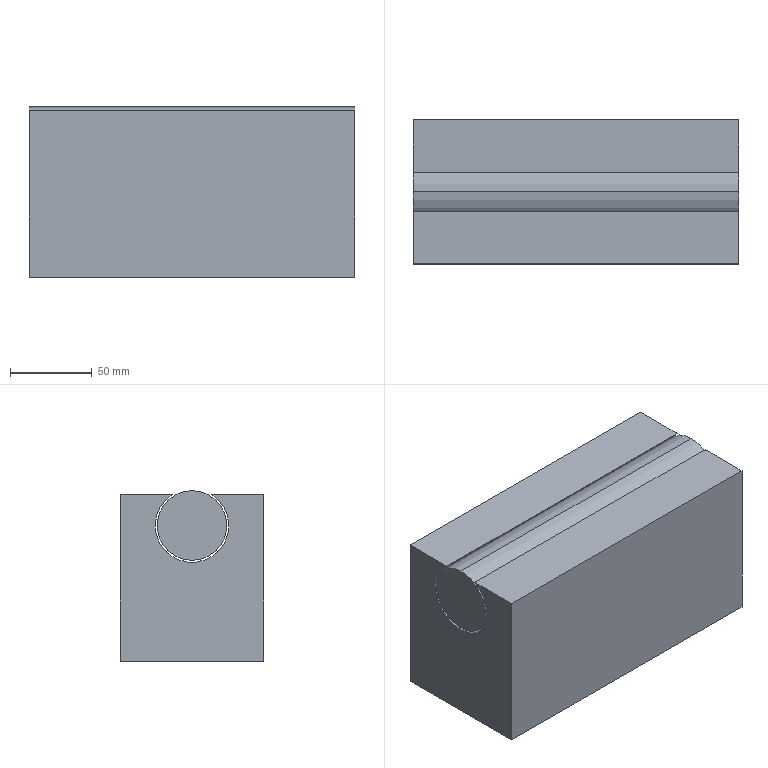Component | SolidWorks | DK1300AInkRollerCoder-1 | 2 solids | 28 faces | box 199 x 88 x 104.3 mm | volume 1763526 mm3 | cylinder 11 | plane 9 | cone 8 | commonest cylinder face diameters 5 x8 42.6 x2 45 x1 | material A3 Steel
build123d program:
from build123d import *

# Parameters (mm, degrees)
SKETCH1_W                  = 88
SKETCH1_H                  = 199
BOSS_EXTRUDE1_DEPTH        = 51
SKETCH2_R                  = 22.5
CUT_EXTRUDE1_DEPTH         = 211.09
SKETCH3_R                  = 21.3
BOSS_EXTRUDE2_DEPTH        = 199
M6_TAPPED_HOLE1_AT_2_COUNT = 2
M6_TAPPED_HOLE1_AT_2_PITCH = 32
M6_TAPPED_HOLE1_AT_3_COUNT = 2
M6_TAPPED_HOLE1_AT_3_PITCH = 62.769
M6_TAPPED_HOLE1_AT_4_COUNT = 2
M6_TAPPED_HOLE1_AT_4_PITCH = 54


with BuildPart() as part:
    # Sketch1 → Boss-Extrude1 (new, symmetric)
    with BuildSketch(Plane.XY):
        Rectangle(SKETCH1_W, SKETCH1_H)
    extrude(amount=BOSS_EXTRUDE1_DEPTH, both=True)

    # Sketch2 → Cut-Extrude1 (cut, through all)
    with BuildSketch(Plane(origin=(0, 99.5, 0), x_dir=(1, 0, 0), z_dir=(0, 1, 0))):
        with Locations((0, -32)):
            Circle(SKETCH2_R)
    extrude(amount=-CUT_EXTRUDE1_DEPTH, mode=Mode.SUBTRACT)

    # Sketch6 → M6 Tapped Hole1 (revolve, cut)
    with BuildSketch(Plane(origin=(16, -5.5, -51), x_dir=(0, 1, 0), z_dir=(1, 0, 0))):
        Polygon((0, 0), (0, 16.502), (2.5, 15), (2.5, 0), align=None)
    m6_tapped_hole1 = revolve(axis=Axis((16, -5.5, -57.35), (0, 0, 1)), mode=Mode.SUBTRACT)

    # M6 Tapped Hole1 at 2: M6 Tapped Hole1 ×2
    with Locations(*[(-i * M6_TAPPED_HOLE1_AT_2_PITCH, 0, 0) for i in range(1, M6_TAPPED_HOLE1_AT_2_COUNT)]):
        add(m6_tapped_hole1, mode=Mode.SUBTRACT)

    # M6 Tapped Hole1 at 3: M6 Tapped Hole1 ×2
    with Locations(*[Vector(-0.5098, -0.8603, 0) * (i * M6_TAPPED_HOLE1_AT_3_PITCH) for i in range(1, M6_TAPPED_HOLE1_AT_3_COUNT)]):
        add(m6_tapped_hole1, mode=Mode.SUBTRACT)

    # M6 Tapped Hole1 at 4: M6 Tapped Hole1 ×2
    with Locations(*[(0, -i * M6_TAPPED_HOLE1_AT_4_PITCH, 0) for i in range(1, M6_TAPPED_HOLE1_AT_4_COUNT)]):
        add(m6_tapped_hole1, mode=Mode.SUBTRACT)


with BuildPart() as body_2:
    # Sketch3 → Boss-Extrude2 (new body)
    with BuildSketch(Plane(origin=(0, 99.5, 0), x_dir=(1, 0, 0), z_dir=(0, 1, 0))):
        with Locations(Location((0, -32, 0), (0, 0, 270))):
            Circle(SKETCH3_R)
    extrude(amount=-BOSS_EXTRUDE2_DEPTH)


solid = Compound([part.part, body_2.part])

# Placed as in the assembly
solid = solid.moved(Location((-212.032, 2.41, -79), (0, 0, 90)))
STEP:
#1=CARTESIAN_POINT('',(-4.43,0.0949,-2.689));
#2=VERTEX_POINT('',#1);
#3=CARTESIAN_POINT('',(-4.43,0.0949,-1.012));
#4=VERTEX_POINT('',#3);
#5=CARTESIAN_POINT('',(-4.43,0.0949,-1.85));
#6=DIRECTION('',(1.,0.,0.));
#7=DIRECTION('',(0.,0.,1.));
#8=AXIS2_PLACEMENT_3D('',#5,#6,#7);
#9=CIRCLE('',#8,0.8386);
#10=EDGE_CURVE('',#2,#4,#9,.T.);
#11=ORIENTED_EDGE('',*,*,#10,.F.);
#12=CARTESIAN_POINT('',(-12.265,0.0949,-2.689));
#13=VERTEX_POINT('',#12);
#14=CARTESIAN_POINT('',(-2.059,0.0949,-2.689));
#15=DIRECTION('',(-1.,-0.,-0.));
#16=VECTOR('',#15,39.37);
#17=LINE('',#14,#16);
#18=EDGE_CURVE('',#2,#13,#17,.T.);
#19=ORIENTED_EDGE('',*,*,#18,.T.);
#20=CARTESIAN_POINT('',(-12.265,0.0949,-1.012));
#21=VERTEX_POINT('',#20);
#22=CARTESIAN_POINT('',(-12.265,0.0949,-1.85));
#23=DIRECTION('',(-1.,-0.,-0.));
#24=DIRECTION('',(0.,-0.,1.));
#25=AXIS2_PLACEMENT_3D('',#22,#23,#24);
#26=CIRCLE('',#25,0.8386);
#27=EDGE_CURVE('',#21,#13,#26,.T.);
#28=ORIENTED_EDGE('',*,*,#27,.F.);
#29=CARTESIAN_POINT('',(-2.059,0.0949,-1.012));
#30=DIRECTION('',(-1.,-0.,-0.));
#31=VECTOR('',#30,39.37);
#32=LINE('',#29,#31);
#33=EDGE_CURVE('',#4,#21,#32,.T.);
#34=ORIENTED_EDGE('',*,*,#33,.F.);
#35=EDGE_LOOP('',(#11,#19,#28,#34));
#36=FACE_OUTER_BOUND('',#35,.T.);
#37=CARTESIAN_POINT('',(-2.059,0.0949,-1.85));
#38=DIRECTION('',(-1.,-0.,-0.));
#39=DIRECTION('',(-0.,-0.,1.));
#40=AXIS2_PLACEMENT_3D('',#37,#38,#39);
#41=CYLINDRICAL_SURFACE('',#40,0.8386);
#42=ADVANCED_FACE('',(#36),#41,.T.);
#43=ORIENTED_EDGE('',*,*,#18,.F.);
#44=CARTESIAN_POINT('',(-4.43,0.0949,-1.85));
#45=DIRECTION('',(1.,0.,0.));
#46=DIRECTION('',(0.,-0.,1.));
#47=AXIS2_PLACEMENT_3D('',#44,#45,#46);
#48=CIRCLE('',#47,0.8386);
#49=EDGE_CURVE('',#4,#2,#48,.T.);
#50=ORIENTED_EDGE('',*,*,#49,.F.);
#51=ORIENTED_EDGE('',*,*,#33,.T.);
#52=CARTESIAN_POINT('',(-12.265,0.0949,-1.85));
#53=DIRECTION('',(-1.,-0.,-0.));
#54=DIRECTION('',(0.,-0.,1.));
#55=AXIS2_PLACEMENT_3D('',#52,#53,#54);
#56=CIRCLE('',#55,0.8386);
#57=EDGE_CURVE('',#13,#21,#56,.T.);
#58=ORIENTED_EDGE('',*,*,#57,.F.);
#59=EDGE_LOOP('',(#43,#50,#51,#58));
#60=FACE_OUTER_BOUND('',#59,.T.);
#61=CARTESIAN_POINT('',(-2.059,0.0949,-1.85));
#62=DIRECTION('',(-1.,-0.,-0.));
#63=DIRECTION('',(-0.,-0.,1.));
#64=AXIS2_PLACEMENT_3D('',#61,#62,#63);
#65=CYLINDRICAL_SURFACE('',#64,0.8386);
#66=ADVANCED_FACE('',(#60),#65,.T.);
#67=ORIENTED_EDGE('',*,*,#27,.T.);
#68=ORIENTED_EDGE('',*,*,#57,.T.);
#69=EDGE_LOOP('',(#67,#68));
#70=FACE_OUTER_BOUND('',#69,.T.);
#71=CARTESIAN_POINT('',(-12.265,0.0949,-1.85));
#72=DIRECTION('',(-1.,-0.,-0.));
#73=DIRECTION('',(-0.,-0.,1.));
#74=AXIS2_PLACEMENT_3D('',#71,#72,#73);
#75=PLANE('',#74);
#76=ADVANCED_FACE('',(#70),#75,.T.);
#77=ORIENTED_EDGE('',*,*,#49,.T.);
#78=ORIENTED_EDGE('',*,*,#10,.T.);
#79=EDGE_LOOP('',(#77,#78));
#80=FACE_OUTER_BOUND('',#79,.T.);
#81=CARTESIAN_POINT('',(-4.43,-1.637,-1.102));
#82=DIRECTION('',(-1.,-0.,-0.));
#83=DIRECTION('',(-0.,-0.,1.));
#84=AXIS2_PLACEMENT_3D('',#81,#82,#83);
#85=PLANE('',#84);
#86=ADVANCED_FACE('',(#80),#85,.F.);
#87=CLOSED_SHELL('',(#42,#66,#76,#86));
#88=MANIFOLD_SOLID_BREP('',#87);
#89=CARTESIAN_POINT('',(-8.131,0.8232,-4.528));
#90=VERTEX_POINT('',#89);
#91=CARTESIAN_POINT('',(-8.131,0.6264,-4.528));
#92=VERTEX_POINT('',#91);
#93=CARTESIAN_POINT('',(-8.131,0.7248,-4.528));
#94=DIRECTION('',(0.,0.,-1.));
#95=DIRECTION('',(0.,-1.,0.));
#96=AXIS2_PLACEMENT_3D('',#93,#94,#95);
#97=CIRCLE('',#96,0.09843);
#98=EDGE_CURVE('',#90,#92,#97,.T.);
#99=ORIENTED_EDGE('',*,*,#98,.F.);
#100=CARTESIAN_POINT('',(-8.131,0.8232,-5.118));
#101=VERTEX_POINT('',#100);
#102=CARTESIAN_POINT('',(-8.131,0.8232,-5.118));
#103=DIRECTION('',(0.,0.,-1.));
#104=VECTOR('',#103,39.37);
#105=LINE('',#102,#104);
#106=EDGE_CURVE('',#90,#101,#105,.T.);
#107=ORIENTED_EDGE('',*,*,#106,.T.);
#108=CARTESIAN_POINT('',(-8.131,0.6264,-5.118));
#109=VERTEX_POINT('',#108);
#110=CARTESIAN_POINT('',(-8.131,0.7248,-5.118));
#111=DIRECTION('',(0.,0.,-1.));
#112=DIRECTION('',(0.,-1.,0.));
#113=AXIS2_PLACEMENT_3D('',#110,#111,#112);
#114=CIRCLE('',#113,0.09843);
#115=EDGE_CURVE('',#101,#109,#114,.T.);
#116=ORIENTED_EDGE('',*,*,#115,.T.);
#117=CARTESIAN_POINT('',(-8.131,0.6264,-5.118));
#118=DIRECTION('',(0.,0.,-1.));
#119=VECTOR('',#118,39.37);
#120=LINE('',#117,#119);
#121=EDGE_CURVE('',#92,#109,#120,.T.);
#122=ORIENTED_EDGE('',*,*,#121,.F.);
#123=EDGE_LOOP('',(#99,#107,#116,#122));
#124=FACE_OUTER_BOUND('',#123,.T.);
#125=CARTESIAN_POINT('',(-8.131,0.7248,-5.118));
#126=DIRECTION('',(0.,0.,-1.));
#127=DIRECTION('',(0.,-1.,0.));
#128=AXIS2_PLACEMENT_3D('',#125,#126,#127);
#129=CYLINDRICAL_SURFACE('',#128,0.09843);
#130=ADVANCED_FACE('',(#124),#129,.F.);
#131=CARTESIAN_POINT('',(-8.131,0.7248,-4.468));
#132=VERTEX_POINT('',#131);
#133=CARTESIAN_POINT('',(-8.131,0.6264,-4.528));
#134=DIRECTION('',(0.,-0.8572,-0.515));
#135=VECTOR('',#134,39.37);
#136=LINE('',#133,#135);
#137=EDGE_CURVE('',#132,#92,#136,.T.);
#138=ORIENTED_EDGE('',*,*,#137,.F.);
#139=CARTESIAN_POINT('',(-8.131,0.8232,-4.528));
#140=DIRECTION('',(-0.,0.8572,-0.515));
#141=VECTOR('',#140,39.37);
#142=LINE('',#139,#141);
#143=EDGE_CURVE('',#132,#90,#142,.T.);
#144=ORIENTED_EDGE('',*,*,#143,.T.);
#145=ORIENTED_EDGE('',*,*,#98,.T.);
#146=EDGE_LOOP('',(#138,#144,#145));
#147=FACE_OUTER_BOUND('',#146,.T.);
#148=CARTESIAN_POINT('',(-8.131,0.7248,-4.528));
#149=DIRECTION('',(0.,0.,-1.));
#150=DIRECTION('',(0.,-1.,0.));
#151=AXIS2_PLACEMENT_3D('',#148,#149,#150);
#152=CONICAL_SURFACE('',#151,0.09843,1.03);
#153=ADVANCED_FACE('',(#147),#152,.F.);
#154=CARTESIAN_POINT('',(-8.131,-0.4366,-4.528));
#155=VERTEX_POINT('',#154);
#156=CARTESIAN_POINT('',(-8.131,-0.6334,-4.528));
#157=VERTEX_POINT('',#156);
#158=CARTESIAN_POINT('',(-8.131,-0.535,-4.528));
#159=DIRECTION('',(0.,0.,-1.));
#160=DIRECTION('',(0.,-1.,0.));
#161=AXIS2_PLACEMENT_3D('',#158,#159,#160);
#162=CIRCLE('',#161,0.09843);
#163=EDGE_CURVE('',#155,#157,#162,.T.);
#164=ORIENTED_EDGE('',*,*,#163,.F.);
#165=CARTESIAN_POINT('',(-8.131,-0.4366,-5.118));
#166=VERTEX_POINT('',#165);
#167=CARTESIAN_POINT('',(-8.131,-0.4366,-5.118));
#168=DIRECTION('',(0.,0.,-1.));
#169=VECTOR('',#168,39.37);
#170=LINE('',#167,#169);
#171=EDGE_CURVE('',#155,#166,#170,.T.);
#172=ORIENTED_EDGE('',*,*,#171,.T.);
#173=CARTESIAN_POINT('',(-8.131,-0.6334,-5.118));
#174=VERTEX_POINT('',#173);
#175=CARTESIAN_POINT('',(-8.131,-0.535,-5.118));
#176=DIRECTION('',(0.,0.,-1.));
#177=DIRECTION('',(0.,-1.,0.));
#178=AXIS2_PLACEMENT_3D('',#175,#176,#177);
#179=CIRCLE('',#178,0.09843);
#180=EDGE_CURVE('',#166,#174,#179,.T.);
#181=ORIENTED_EDGE('',*,*,#180,.T.);
#182=CARTESIAN_POINT('',(-8.131,-0.6334,-5.118));
#183=DIRECTION('',(0.,0.,-1.));
#184=VECTOR('',#183,39.37);
#185=LINE('',#182,#184);
#186=EDGE_CURVE('',#157,#174,#185,.T.);
#187=ORIENTED_EDGE('',*,*,#186,.F.);
#188=EDGE_LOOP('',(#164,#172,#181,#187));
#189=FACE_OUTER_BOUND('',#188,.T.);
#190=CARTESIAN_POINT('',(-8.131,-0.535,-5.118));
#191=DIRECTION('',(0.,0.,-1.));
#192=DIRECTION('',(0.,-1.,0.));
#193=AXIS2_PLACEMENT_3D('',#190,#191,#192);
#194=CYLINDRICAL_SURFACE('',#193,0.09843);
#195=ADVANCED_FACE('',(#189),#194,.F.);
#196=CARTESIAN_POINT('',(-8.131,-0.535,-4.468));
#197=VERTEX_POINT('',#196);
#198=CARTESIAN_POINT('',(-8.131,-0.6334,-4.528));
#199=DIRECTION('',(0.,-0.8572,-0.515));
#200=VECTOR('',#199,39.37);
#201=LINE('',#198,#200);
#202=EDGE_CURVE('',#197,#157,#201,.T.);
#203=ORIENTED_EDGE('',*,*,#202,.F.);
#204=CARTESIAN_POINT('',(-8.131,-0.4366,-4.528));
#205=DIRECTION('',(-0.,0.8572,-0.515));
#206=VECTOR('',#205,39.37);
#207=LINE('',#204,#206);
#208=EDGE_CURVE('',#197,#155,#207,.T.);
#209=ORIENTED_EDGE('',*,*,#208,.T.);
#210=ORIENTED_EDGE('',*,*,#163,.T.);
#211=EDGE_LOOP('',(#203,#209,#210));
#212=FACE_OUTER_BOUND('',#211,.T.);
#213=CARTESIAN_POINT('',(-8.131,-0.535,-4.528));
#214=DIRECTION('',(0.,0.,-1.));
#215=DIRECTION('',(0.,-1.,0.));
#216=AXIS2_PLACEMENT_3D('',#213,#214,#215);
#217=CONICAL_SURFACE('',#216,0.09843,1.03);
#218=ADVANCED_FACE('',(#212),#217,.F.);
#219=CARTESIAN_POINT('',(-6.005,-0.4366,-4.528));
#220=VERTEX_POINT('',#219);
#221=CARTESIAN_POINT('',(-6.005,-0.6334,-4.528));
#222=VERTEX_POINT('',#221);
#223=CARTESIAN_POINT('',(-6.005,-0.535,-4.528));
#224=DIRECTION('',(0.,0.,-1.));
#225=DIRECTION('',(0.,-1.,0.));
#226=AXIS2_PLACEMENT_3D('',#223,#224,#225);
#227=CIRCLE('',#226,0.09843);
#228=EDGE_CURVE('',#220,#222,#227,.T.);
#229=ORIENTED_EDGE('',*,*,#228,.F.);
#230=CARTESIAN_POINT('',(-6.005,-0.4366,-5.118));
#231=VERTEX_POINT('',#230);
#232=CARTESIAN_POINT('',(-6.005,-0.4366,-5.118));
#233=DIRECTION('',(0.,0.,-1.));
#234=VECTOR('',#233,39.37);
#235=LINE('',#232,#234);
#236=EDGE_CURVE('',#220,#231,#235,.T.);
#237=ORIENTED_EDGE('',*,*,#236,.T.);
#238=CARTESIAN_POINT('',(-6.005,-0.6334,-5.118));
#239=VERTEX_POINT('',#238);
#240=CARTESIAN_POINT('',(-6.005,-0.535,-5.118));
#241=DIRECTION('',(0.,0.,-1.));
#242=DIRECTION('',(0.,-1.,0.));
#243=AXIS2_PLACEMENT_3D('',#240,#241,#242);
#244=CIRCLE('',#243,0.09843);
#245=EDGE_CURVE('',#231,#239,#244,.T.);
#246=ORIENTED_EDGE('',*,*,#245,.T.);
#247=CARTESIAN_POINT('',(-6.005,-0.6334,-5.118));
#248=DIRECTION('',(0.,0.,-1.));
#249=VECTOR('',#248,39.37);
#250=LINE('',#247,#249);
#251=EDGE_CURVE('',#222,#239,#250,.T.);
#252=ORIENTED_EDGE('',*,*,#251,.F.);
#253=EDGE_LOOP('',(#229,#237,#246,#252));
#254=FACE_OUTER_BOUND('',#253,.T.);
#255=CARTESIAN_POINT('',(-6.005,-0.535,-5.118));
#256=DIRECTION('',(0.,0.,-1.));
#257=DIRECTION('',(0.,-1.,0.));
#258=AXIS2_PLACEMENT_3D('',#255,#256,#257);
#259=CYLINDRICAL_SURFACE('',#258,0.09843);
#260=ADVANCED_FACE('',(#254),#259,.F.);
#261=CARTESIAN_POINT('',(-6.005,-0.535,-4.468));
#262=VERTEX_POINT('',#261);
#263=CARTESIAN_POINT('',(-6.005,-0.6334,-4.528));
#264=DIRECTION('',(0.,-0.8572,-0.515));
#265=VECTOR('',#264,39.37);
#266=LINE('',#263,#265);
#267=EDGE_CURVE('',#262,#222,#266,.T.);
#268=ORIENTED_EDGE('',*,*,#267,.F.);
#269=CARTESIAN_POINT('',(-6.005,-0.4366,-4.528));
#270=DIRECTION('',(-0.,0.8572,-0.515));
#271=VECTOR('',#270,39.37);
#272=LINE('',#269,#271);
#273=EDGE_CURVE('',#262,#220,#272,.T.);
#274=ORIENTED_EDGE('',*,*,#273,.T.);
#275=ORIENTED_EDGE('',*,*,#228,.T.);
#276=EDGE_LOOP('',(#268,#274,#275));
#277=FACE_OUTER_BOUND('',#276,.T.);
#278=CARTESIAN_POINT('',(-6.005,-0.535,-4.528));
#279=DIRECTION('',(0.,0.,-1.));
#280=DIRECTION('',(0.,-1.,0.));
#281=AXIS2_PLACEMENT_3D('',#278,#279,#280);
#282=CONICAL_SURFACE('',#281,0.09843,1.03);
#283=ADVANCED_FACE('',(#277),#282,.F.);
#284=CARTESIAN_POINT('',(-6.005,0.8232,-4.528));
#285=VERTEX_POINT('',#284);
#286=CARTESIAN_POINT('',(-6.005,0.6264,-4.528));
#287=VERTEX_POINT('',#286);
#288=CARTESIAN_POINT('',(-6.005,0.7248,-4.528));
#289=DIRECTION('',(0.,0.,-1.));
#290=DIRECTION('',(0.,-1.,0.));
#291=AXIS2_PLACEMENT_3D('',#288,#289,#290);
#292=CIRCLE('',#291,0.09843);
#293=EDGE_CURVE('',#285,#287,#292,.T.);
#294=ORIENTED_EDGE('',*,*,#293,.F.);
#295=CARTESIAN_POINT('',(-6.005,0.8232,-5.118));
#296=VERTEX_POINT('',#295);
#297=CARTESIAN_POINT('',(-6.005,0.8232,-5.118));
#298=DIRECTION('',(0.,0.,-1.));
#299=VECTOR('',#298,39.37);
#300=LINE('',#297,#299);
#301=EDGE_CURVE('',#285,#296,#300,.T.);
#302=ORIENTED_EDGE('',*,*,#301,.T.);
#303=CARTESIAN_POINT('',(-6.005,0.6264,-5.118));
#304=VERTEX_POINT('',#303);
#305=CARTESIAN_POINT('',(-6.005,0.7248,-5.118));
#306=DIRECTION('',(0.,0.,-1.));
#307=DIRECTION('',(0.,-1.,0.));
#308=AXIS2_PLACEMENT_3D('',#305,#306,#307);
#309=CIRCLE('',#308,0.09843);
#310=EDGE_CURVE('',#296,#304,#309,.T.);
#311=ORIENTED_EDGE('',*,*,#310,.T.);
#312=CARTESIAN_POINT('',(-6.005,0.6264,-5.118));
#313=DIRECTION('',(0.,0.,-1.));
#314=VECTOR('',#313,39.37);
#315=LINE('',#312,#314);
#316=EDGE_CURVE('',#287,#304,#315,.T.);
#317=ORIENTED_EDGE('',*,*,#316,.F.);
#318=EDGE_LOOP('',(#294,#302,#311,#317));
#319=FACE_OUTER_BOUND('',#318,.T.);
#320=CARTESIAN_POINT('',(-6.005,0.7248,-5.118));
#321=DIRECTION('',(0.,0.,-1.));
#322=DIRECTION('',(0.,-1.,0.));
#323=AXIS2_PLACEMENT_3D('',#320,#321,#322);
#324=CYLINDRICAL_SURFACE('',#323,0.09843);
#325=ADVANCED_FACE('',(#319),#324,.F.);
#326=CARTESIAN_POINT('',(-6.005,0.7248,-4.468));
#327=VERTEX_POINT('',#326);
#328=CARTESIAN_POINT('',(-6.005,0.6264,-4.528));
#329=DIRECTION('',(0.,-0.8572,-0.515));
#330=VECTOR('',#329,39.37);
#331=LINE('',#328,#330);
#332=EDGE_CURVE('',#327,#287,#331,.T.);
#333=ORIENTED_EDGE('',*,*,#332,.F.);
#334=CARTESIAN_POINT('',(-6.005,0.8232,-4.528));
#335=DIRECTION('',(-0.,0.8572,-0.515));
#336=VECTOR('',#335,39.37);
#337=LINE('',#334,#336);
#338=EDGE_CURVE('',#327,#285,#337,.T.);
#339=ORIENTED_EDGE('',*,*,#338,.T.);
#340=ORIENTED_EDGE('',*,*,#293,.T.);
#341=EDGE_LOOP('',(#333,#339,#340));
#342=FACE_OUTER_BOUND('',#341,.T.);
#343=CARTESIAN_POINT('',(-6.005,0.7248,-4.528));
#344=DIRECTION('',(0.,0.,-1.));
#345=DIRECTION('',(0.,-1.,0.));
#346=AXIS2_PLACEMENT_3D('',#343,#344,#345);
#347=CONICAL_SURFACE('',#346,0.09843,1.03);
#348=ADVANCED_FACE('',(#342),#347,.F.);
#349=CARTESIAN_POINT('',(-4.43,-1.637,-1.102));
#350=VERTEX_POINT('',#349);
#351=CARTESIAN_POINT('',(-4.43,-0.3796,-1.102));
#352=VERTEX_POINT('',#351);
#353=CARTESIAN_POINT('',(-4.43,-1.637,-1.102));
#354=DIRECTION('',(-0.,1.,0.));
#355=VECTOR('',#354,39.37);
#356=LINE('',#353,#355);
#357=EDGE_CURVE('',#350,#352,#356,.T.);
#358=ORIENTED_EDGE('',*,*,#357,.T.);
#359=CARTESIAN_POINT('',(-12.265,-0.3796,-1.102));
#360=VERTEX_POINT('',#359);
#361=CARTESIAN_POINT('',(-4.43,-0.3796,-1.102));
#362=DIRECTION('',(-1.,-0.,-0.));
#363=VECTOR('',#362,39.37);
#364=LINE('',#361,#363);
#365=EDGE_CURVE('',#352,#360,#364,.T.);
#366=ORIENTED_EDGE('',*,*,#365,.T.);
#367=CARTESIAN_POINT('',(-12.265,-1.637,-1.102));
#368=VERTEX_POINT('',#367);
#369=CARTESIAN_POINT('',(-12.265,-1.637,-1.102));
#370=DIRECTION('',(0.,-1.,-0.));
#371=VECTOR('',#370,39.37);
#372=LINE('',#369,#371);
#373=EDGE_CURVE('',#360,#368,#372,.T.);
#374=ORIENTED_EDGE('',*,*,#373,.T.);
#375=CARTESIAN_POINT('',(-4.43,-1.637,-1.102));
#376=DIRECTION('',(1.,0.,0.));
#377=VECTOR('',#376,39.37);
#378=LINE('',#375,#377);
#379=EDGE_CURVE('',#368,#350,#378,.T.);
#380=ORIENTED_EDGE('',*,*,#379,.T.);
#381=EDGE_LOOP('',(#358,#366,#374,#380));
#382=FACE_OUTER_BOUND('',#381,.T.);
#383=CARTESIAN_POINT('',(-8.348,0.0949,-1.102));
#384=DIRECTION('',(0.,0.,-1.));
#385=DIRECTION('',(0.,-1.,-0.));
#386=AXIS2_PLACEMENT_3D('',#383,#384,#385);
#387=PLANE('',#386);
#388=ADVANCED_FACE('',(#382),#387,.F.);
#389=CARTESIAN_POINT('',(-4.43,1.827,-5.118));
#390=VERTEX_POINT('',#389);
#391=CARTESIAN_POINT('',(-12.265,1.827,-5.118));
#392=VERTEX_POINT('',#391);
#393=CARTESIAN_POINT('',(-4.43,1.827,-5.118));
#394=DIRECTION('',(-1.,-0.,-0.));
#395=VECTOR('',#394,39.37);
#396=LINE('',#393,#395);
#397=EDGE_CURVE('',#390,#392,#396,.T.);
#398=ORIENTED_EDGE('',*,*,#397,.T.);
#399=CARTESIAN_POINT('',(-12.265,1.827,-1.102));
#400=VERTEX_POINT('',#399);
#401=CARTESIAN_POINT('',(-12.265,1.827,-1.102));
#402=DIRECTION('',(0.,0.,-1.));
#403=VECTOR('',#402,39.37);
#404=LINE('',#401,#403);
#405=EDGE_CURVE('',#400,#392,#404,.T.);
#406=ORIENTED_EDGE('',*,*,#405,.F.);
#407=CARTESIAN_POINT('',(-4.43,1.827,-1.102));
#408=VERTEX_POINT('',#407);
#409=CARTESIAN_POINT('',(-4.43,1.827,-1.102));
#410=DIRECTION('',(-1.,-0.,-0.));
#411=VECTOR('',#410,39.37);
#412=LINE('',#409,#411);
#413=EDGE_CURVE('',#408,#400,#412,.T.);
#414=ORIENTED_EDGE('',*,*,#413,.F.);
#415=CARTESIAN_POINT('',(-4.43,1.827,-1.102));
#416=DIRECTION('',(0.,0.,-1.));
#417=VECTOR('',#416,39.37);
#418=LINE('',#415,#417);
#419=EDGE_CURVE('',#408,#390,#418,.T.);
#420=ORIENTED_EDGE('',*,*,#419,.T.);
#421=EDGE_LOOP('',(#398,#406,#414,#420));
#422=FACE_OUTER_BOUND('',#421,.T.);
#423=CARTESIAN_POINT('',(-4.43,1.827,-1.102));
#424=DIRECTION('',(0.,-1.,-0.));
#425=DIRECTION('',(-0.,-0.,1.));
#426=AXIS2_PLACEMENT_3D('',#423,#424,#425);
#427=PLANE('',#426);
#428=ADVANCED_FACE('',(#422),#427,.F.);
#429=ORIENTED_EDGE('',*,*,#373,.F.);
#430=CARTESIAN_POINT('',(-12.265,0.5694,-1.102));
#431=VERTEX_POINT('',#430);
#432=CARTESIAN_POINT('',(-12.265,0.0949,-1.85));
#433=DIRECTION('',(-1.,-0.,-0.));
#434=DIRECTION('',(0.,-0.,1.));
#435=AXIS2_PLACEMENT_3D('',#432,#433,#434);
#436=CIRCLE('',#435,0.8858);
#437=EDGE_CURVE('',#431,#360,#436,.T.);
#438=ORIENTED_EDGE('',*,*,#437,.F.);
#439=CARTESIAN_POINT('',(-12.265,-1.637,-1.102));
#440=DIRECTION('',(0.,-1.,-0.));
#441=VECTOR('',#440,39.37);
#442=LINE('',#439,#441);
#443=EDGE_CURVE('',#400,#431,#442,.T.);
#444=ORIENTED_EDGE('',*,*,#443,.F.);
#445=ORIENTED_EDGE('',*,*,#405,.T.);
#446=CARTESIAN_POINT('',(-12.265,-1.637,-5.118));
#447=VERTEX_POINT('',#446);
#448=CARTESIAN_POINT('',(-12.265,-1.637,-5.118));
#449=DIRECTION('',(0.,-1.,-0.));
#450=VECTOR('',#449,39.37);
#451=LINE('',#448,#450);
#452=EDGE_CURVE('',#392,#447,#451,.T.);
#453=ORIENTED_EDGE('',*,*,#452,.T.);
#454=CARTESIAN_POINT('',(-12.265,-1.637,-1.102));
#455=DIRECTION('',(0.,0.,-1.));
#456=VECTOR('',#455,39.37);
#457=LINE('',#454,#456);
#458=EDGE_CURVE('',#368,#447,#457,.T.);
#459=ORIENTED_EDGE('',*,*,#458,.F.);
#460=EDGE_LOOP('',(#429,#438,#444,#445,#453,#459));
#461=FACE_OUTER_BOUND('',#460,.T.);
#462=CARTESIAN_POINT('',(-12.265,-1.637,-1.102));
#463=DIRECTION('',(1.,0.,0.));
#464=DIRECTION('',(0.,0.,-1.));
#465=AXIS2_PLACEMENT_3D('',#462,#463,#464);
#466=PLANE('',#465);
#467=ADVANCED_FACE('',(#461),#466,.F.);
#468=CARTESIAN_POINT('',(-4.43,-1.637,-5.118));
#469=VERTEX_POINT('',#468);
#470=CARTESIAN_POINT('',(-4.43,-1.637,-5.118));
#471=DIRECTION('',(1.,0.,0.));
#472=VECTOR('',#471,39.37);
#473=LINE('',#470,#472);
#474=EDGE_CURVE('',#447,#469,#473,.T.);
#475=ORIENTED_EDGE('',*,*,#474,.T.);
#476=CARTESIAN_POINT('',(-4.43,-1.637,-1.102));
#477=DIRECTION('',(0.,0.,-1.));
#478=VECTOR('',#477,39.37);
#479=LINE('',#476,#478);
#480=EDGE_CURVE('',#350,#469,#479,.T.);
#481=ORIENTED_EDGE('',*,*,#480,.F.);
#482=ORIENTED_EDGE('',*,*,#379,.F.);
#483=ORIENTED_EDGE('',*,*,#458,.T.);
#484=EDGE_LOOP('',(#475,#481,#482,#483));
#485=FACE_OUTER_BOUND('',#484,.T.);
#486=CARTESIAN_POINT('',(-4.43,-1.637,-1.102));
#487=DIRECTION('',(-0.,1.,0.));
#488=DIRECTION('',(0.,0.,-1.));
#489=AXIS2_PLACEMENT_3D('',#486,#487,#488);
#490=PLANE('',#489);
#491=ADVANCED_FACE('',(#485),#490,.F.);
#492=CARTESIAN_POINT('',(-4.43,0.5694,-1.102));
#493=VERTEX_POINT('',#492);
#494=CARTESIAN_POINT('',(-4.43,-1.637,-1.102));
#495=DIRECTION('',(-0.,1.,0.));
#496=VECTOR('',#495,39.37);
#497=LINE('',#494,#496);
#498=EDGE_CURVE('',#493,#408,#497,.T.);
#499=ORIENTED_EDGE('',*,*,#498,.F.);
#500=CARTESIAN_POINT('',(-4.43,0.0949,-1.85));
#501=DIRECTION('',(-1.,-0.,-0.));
#502=DIRECTION('',(0.,-0.,1.));
#503=AXIS2_PLACEMENT_3D('',#500,#501,#502);
#504=CIRCLE('',#503,0.8858);
#505=EDGE_CURVE('',#493,#352,#504,.T.);
#506=ORIENTED_EDGE('',*,*,#505,.T.);
#507=ORIENTED_EDGE('',*,*,#357,.F.);
#508=ORIENTED_EDGE('',*,*,#480,.T.);
#509=CARTESIAN_POINT('',(-4.43,-1.637,-5.118));
#510=DIRECTION('',(-0.,1.,0.));
#511=VECTOR('',#510,39.37);
#512=LINE('',#509,#511);
#513=EDGE_CURVE('',#469,#390,#512,.T.);
#514=ORIENTED_EDGE('',*,*,#513,.T.);
#515=ORIENTED_EDGE('',*,*,#419,.F.);
#516=EDGE_LOOP('',(#499,#506,#507,#508,#514,#515));
#517=FACE_OUTER_BOUND('',#516,.T.);
#518=CARTESIAN_POINT('',(-4.43,-1.637,-1.102));
#519=DIRECTION('',(-1.,-0.,-0.));
#520=DIRECTION('',(-0.,-0.,1.));
#521=AXIS2_PLACEMENT_3D('',#518,#519,#520);
#522=PLANE('',#521);
#523=ADVANCED_FACE('',(#517),#522,.F.);
#524=ORIENTED_EDGE('',*,*,#443,.T.);
#525=CARTESIAN_POINT('',(-4.43,0.5694,-1.102));
#526=DIRECTION('',(1.,0.,0.));
#527=VECTOR('',#526,39.37);
#528=LINE('',#525,#527);
#529=EDGE_CURVE('',#431,#493,#528,.T.);
#530=ORIENTED_EDGE('',*,*,#529,.T.);
#531=ORIENTED_EDGE('',*,*,#498,.T.);
#532=ORIENTED_EDGE('',*,*,#413,.T.);
#533=EDGE_LOOP('',(#524,#530,#531,#532));
#534=FACE_OUTER_BOUND('',#533,.T.);
#535=CARTESIAN_POINT('',(-8.348,0.0949,-1.102));
#536=DIRECTION('',(0.,0.,-1.));
#537=DIRECTION('',(0.,-1.,-0.));
#538=AXIS2_PLACEMENT_3D('',#535,#536,#537);
#539=PLANE('',#538);
#540=ADVANCED_FACE('',(#534),#539,.F.);
#541=CARTESIAN_POINT('',(-8.131,0.7248,-5.118));
#542=DIRECTION('',(0.,0.,-1.));
#543=DIRECTION('',(0.,-1.,0.));
#544=AXIS2_PLACEMENT_3D('',#541,#542,#543);
#545=CIRCLE('',#544,0.09843);
#546=EDGE_CURVE('',#109,#101,#545,.T.);
#547=ORIENTED_EDGE('',*,*,#546,.F.);
#548=ORIENTED_EDGE('',*,*,#115,.F.);
#549=EDGE_LOOP('',(#547,#548));
#550=FACE_BOUND('',#549,.T.);
#551=CARTESIAN_POINT('',(-8.131,-0.535,-5.118));
#552=DIRECTION('',(0.,0.,-1.));
#553=DIRECTION('',(0.,-1.,0.));
#554=AXIS2_PLACEMENT_3D('',#551,#552,#553);
#555=CIRCLE('',#554,0.09843);
#556=EDGE_CURVE('',#174,#166,#555,.T.);
#557=ORIENTED_EDGE('',*,*,#556,.F.);
#558=ORIENTED_EDGE('',*,*,#180,.F.);
#559=EDGE_LOOP('',(#557,#558));
#560=FACE_BOUND('',#559,.T.);
#561=CARTESIAN_POINT('',(-6.005,-0.535,-5.118));
#562=DIRECTION('',(0.,0.,-1.));
#563=DIRECTION('',(0.,-1.,0.));
#564=AXIS2_PLACEMENT_3D('',#561,#562,#563);
#565=CIRCLE('',#564,0.09843);
#566=EDGE_CURVE('',#239,#231,#565,.T.);
#567=ORIENTED_EDGE('',*,*,#566,.F.);
#568=ORIENTED_EDGE('',*,*,#245,.F.);
#569=EDGE_LOOP('',(#567,#568));
#570=FACE_BOUND('',#569,.T.);
#571=CARTESIAN_POINT('',(-6.005,0.7248,-5.118));
#572=DIRECTION('',(0.,0.,-1.));
#573=DIRECTION('',(0.,-1.,0.));
#574=AXIS2_PLACEMENT_3D('',#571,#572,#573);
#575=CIRCLE('',#574,0.09843);
#576=EDGE_CURVE('',#304,#296,#575,.T.);
#577=ORIENTED_EDGE('',*,*,#576,.F.);
#578=ORIENTED_EDGE('',*,*,#310,.F.);
#579=EDGE_LOOP('',(#577,#578));
#580=FACE_BOUND('',#579,.T.);
#581=ORIENTED_EDGE('',*,*,#397,.F.);
#582=ORIENTED_EDGE('',*,*,#513,.F.);
#583=ORIENTED_EDGE('',*,*,#474,.F.);
#584=ORIENTED_EDGE('',*,*,#452,.F.);
#585=EDGE_LOOP('',(#581,#582,#583,#584));
#586=FACE_OUTER_BOUND('',#585,.T.);
#587=CARTESIAN_POINT('',(-8.348,0.0949,-5.118));
#588=DIRECTION('',(0.,0.,-1.));
#589=DIRECTION('',(0.,-1.,-0.));
#590=AXIS2_PLACEMENT_3D('',#587,#588,#589);
#591=PLANE('',#590);
#592=ADVANCED_FACE('',(#550,#560,#570,#580,#586),#591,.T.);
#593=ORIENTED_EDGE('',*,*,#505,.F.);
#594=ORIENTED_EDGE('',*,*,#529,.F.);
#595=ORIENTED_EDGE('',*,*,#437,.T.);
#596=ORIENTED_EDGE('',*,*,#365,.F.);
#597=EDGE_LOOP('',(#593,#594,#595,#596));
#598=FACE_OUTER_BOUND('',#597,.T.);
#599=CARTESIAN_POINT('',(-4.43,0.0949,-1.85));
#600=DIRECTION('',(-1.,-0.,-0.));
#601=DIRECTION('',(0.,-0.,1.));
#602=AXIS2_PLACEMENT_3D('',#599,#600,#601);
#603=CYLINDRICAL_SURFACE('',#602,0.8858);
#604=ADVANCED_FACE('',(#598),#603,.F.);
#605=ORIENTED_EDGE('',*,*,#338,.F.);
#606=ORIENTED_EDGE('',*,*,#332,.T.);
#607=CARTESIAN_POINT('',(-6.005,0.7248,-4.528));
#608=DIRECTION('',(0.,0.,-1.));
#609=DIRECTION('',(0.,-1.,0.));
#610=AXIS2_PLACEMENT_3D('',#607,#608,#609);
#611=CIRCLE('',#610,0.09843);
#612=EDGE_CURVE('',#287,#285,#611,.T.);
#613=ORIENTED_EDGE('',*,*,#612,.T.);
#614=EDGE_LOOP('',(#605,#606,#613));
#615=FACE_OUTER_BOUND('',#614,.T.);
#616=CARTESIAN_POINT('',(-6.005,0.7248,-4.528));
#617=DIRECTION('',(0.,0.,-1.));
#618=DIRECTION('',(0.,-1.,0.));
#619=AXIS2_PLACEMENT_3D('',#616,#617,#618);
#620=CONICAL_SURFACE('',#619,0.09843,1.03);
#621=ADVANCED_FACE('',(#615),#620,.F.);
#622=ORIENTED_EDGE('',*,*,#301,.F.);
#623=ORIENTED_EDGE('',*,*,#612,.F.);
#624=ORIENTED_EDGE('',*,*,#316,.T.);
#625=ORIENTED_EDGE('',*,*,#576,.T.);
#626=EDGE_LOOP('',(#622,#623,#624,#625));
#627=FACE_OUTER_BOUND('',#626,.T.);
#628=CARTESIAN_POINT('',(-6.005,0.7248,-5.118));
#629=DIRECTION('',(0.,0.,-1.));
#630=DIRECTION('',(0.,-1.,0.));
#631=AXIS2_PLACEMENT_3D('',#628,#629,#630);
#632=CYLINDRICAL_SURFACE('',#631,0.09843);
#633=ADVANCED_FACE('',(#627),#632,.F.);
#634=ORIENTED_EDGE('',*,*,#273,.F.);
#635=ORIENTED_EDGE('',*,*,#267,.T.);
#636=CARTESIAN_POINT('',(-6.005,-0.535,-4.528));
#637=DIRECTION('',(0.,0.,-1.));
#638=DIRECTION('',(0.,-1.,0.));
#639=AXIS2_PLACEMENT_3D('',#636,#637,#638);
#640=CIRCLE('',#639,0.09843);
#641=EDGE_CURVE('',#222,#220,#640,.T.);
#642=ORIENTED_EDGE('',*,*,#641,.T.);
#643=EDGE_LOOP('',(#634,#635,#642));
#644=FACE_OUTER_BOUND('',#643,.T.);
#645=CARTESIAN_POINT('',(-6.005,-0.535,-4.528));
#646=DIRECTION('',(0.,0.,-1.));
#647=DIRECTION('',(0.,-1.,0.));
#648=AXIS2_PLACEMENT_3D('',#645,#646,#647);
#649=CONICAL_SURFACE('',#648,0.09843,1.03);
#650=ADVANCED_FACE('',(#644),#649,.F.);
#651=ORIENTED_EDGE('',*,*,#236,.F.);
#652=ORIENTED_EDGE('',*,*,#641,.F.);
#653=ORIENTED_EDGE('',*,*,#251,.T.);
#654=ORIENTED_EDGE('',*,*,#566,.T.);
#655=EDGE_LOOP('',(#651,#652,#653,#654));
#656=FACE_OUTER_BOUND('',#655,.T.);
#657=CARTESIAN_POINT('',(-6.005,-0.535,-5.118));
#658=DIRECTION('',(0.,0.,-1.));
#659=DIRECTION('',(0.,-1.,0.));
#660=AXIS2_PLACEMENT_3D('',#657,#658,#659);
#661=CYLINDRICAL_SURFACE('',#660,0.09843);
#662=ADVANCED_FACE('',(#656),#661,.F.);
#663=ORIENTED_EDGE('',*,*,#208,.F.);
#664=ORIENTED_EDGE('',*,*,#202,.T.);
#665=CARTESIAN_POINT('',(-8.131,-0.535,-4.528));
#666=DIRECTION('',(0.,0.,-1.));
#667=DIRECTION('',(0.,-1.,0.));
#668=AXIS2_PLACEMENT_3D('',#665,#666,#667);
#669=CIRCLE('',#668,0.09843);
#670=EDGE_CURVE('',#157,#155,#669,.T.);
#671=ORIENTED_EDGE('',*,*,#670,.T.);
#672=EDGE_LOOP('',(#663,#664,#671));
#673=FACE_OUTER_BOUND('',#672,.T.);
#674=CARTESIAN_POINT('',(-8.131,-0.535,-4.528));
#675=DIRECTION('',(0.,0.,-1.));
#676=DIRECTION('',(0.,-1.,0.));
#677=AXIS2_PLACEMENT_3D('',#674,#675,#676);
#678=CONICAL_SURFACE('',#677,0.09843,1.03);
#679=ADVANCED_FACE('',(#673),#678,.F.);
#680=ORIENTED_EDGE('',*,*,#171,.F.);
#681=ORIENTED_EDGE('',*,*,#670,.F.);
#682=ORIENTED_EDGE('',*,*,#186,.T.);
#683=ORIENTED_EDGE('',*,*,#556,.T.);
#684=EDGE_LOOP('',(#680,#681,#682,#683));
#685=FACE_OUTER_BOUND('',#684,.T.);
#686=CARTESIAN_POINT('',(-8.131,-0.535,-5.118));
#687=DIRECTION('',(0.,0.,-1.));
#688=DIRECTION('',(0.,-1.,0.));
#689=AXIS2_PLACEMENT_3D('',#686,#687,#688);
#690=CYLINDRICAL_SURFACE('',#689,0.09843);
#691=ADVANCED_FACE('',(#685),#690,.F.);
#692=ORIENTED_EDGE('',*,*,#143,.F.);
#693=ORIENTED_EDGE('',*,*,#137,.T.);
#694=CARTESIAN_POINT('',(-8.131,0.7248,-4.528));
#695=DIRECTION('',(0.,0.,-1.));
#696=DIRECTION('',(0.,-1.,0.));
#697=AXIS2_PLACEMENT_3D('',#694,#695,#696);
#698=CIRCLE('',#697,0.09843);
#699=EDGE_CURVE('',#92,#90,#698,.T.);
#700=ORIENTED_EDGE('',*,*,#699,.T.);
#701=EDGE_LOOP('',(#692,#693,#700));
#702=FACE_OUTER_BOUND('',#701,.T.);
#703=CARTESIAN_POINT('',(-8.131,0.7248,-4.528));
#704=DIRECTION('',(0.,0.,-1.));
#705=DIRECTION('',(0.,-1.,0.));
#706=AXIS2_PLACEMENT_3D('',#703,#704,#705);
#707=CONICAL_SURFACE('',#706,0.09843,1.03);
#708=ADVANCED_FACE('',(#702),#707,.F.);
#709=ORIENTED_EDGE('',*,*,#106,.F.);
#710=ORIENTED_EDGE('',*,*,#699,.F.);
#711=ORIENTED_EDGE('',*,*,#121,.T.);
#712=ORIENTED_EDGE('',*,*,#546,.T.);
#713=EDGE_LOOP('',(#709,#710,#711,#712));
#714=FACE_OUTER_BOUND('',#713,.T.);
#715=CARTESIAN_POINT('',(-8.131,0.7248,-5.118));
#716=DIRECTION('',(0.,0.,-1.));
#717=DIRECTION('',(0.,-1.,0.));
#718=AXIS2_PLACEMENT_3D('',#715,#716,#717);
#719=CYLINDRICAL_SURFACE('',#718,0.09843);
#720=ADVANCED_FACE('',(#714),#719,.F.);
#721=CLOSED_SHELL('',(#130,#153,#195,#218,#260,#283,#325,#348,#388,#428,#467,#491,#523,#540,#592,#604,#621,#633,#650,#662,#679,#691,#708,#720));
#722=MANIFOLD_SOLID_BREP('',#721);
#723=CARTESIAN_POINT('',(0.,0.,0.));
#724=DIRECTION('',(0.,0.,1.));
#725=DIRECTION('',(1.,0.,0.));
#726=AXIS2_PLACEMENT_3D('',#723,#724,#725);
#727=(LENGTH_UNIT()NAMED_UNIT(*)SI_UNIT($,.METRE.));
#728=LENGTH_MEASURE_WITH_UNIT(LENGTH_MEASURE(0.0254),#727);
#729=DIMENSIONAL_EXPONENTS(1.,0.,0.,0.,0.,0.,0.);
#730=(CONVERSION_BASED_UNIT('',#728)LENGTH_UNIT()NAMED_UNIT(#729));
#731=UNCERTAINTY_MEASURE_WITH_UNIT(LENGTH_MEASURE(0.00001),#730,'','');
#732=(NAMED_UNIT(*)PLANE_ANGLE_UNIT()SI_UNIT($,.RADIAN.));
#733=(NAMED_UNIT(*)SI_UNIT($,.STERADIAN.)SOLID_ANGLE_UNIT());
#734=(GEOMETRIC_REPRESENTATION_CONTEXT(3)GLOBAL_UNCERTAINTY_ASSIGNED_CONTEXT((#731))GLOBAL_UNIT_ASSIGNED_CONTEXT((#730,#732,#733))REPRESENTATION_CONTEXT('',''));
#735=ADVANCED_BREP_SHAPE_REPRESENTATION('',(#88,#722,#726),#734);
#736=COLOUR_RGB('',0.7922,0.8196,0.9333);
#737=FILL_AREA_STYLE_COLOUR('',#736);
#738=FILL_AREA_STYLE('',(#737));
#739=SURFACE_STYLE_FILL_AREA(#738);
#740=SURFACE_SIDE_STYLE('',(#739));
#741=SURFACE_STYLE_USAGE(.BOTH.,#740);
#742=PRESENTATION_STYLE_ASSIGNMENT((#741));
#743=STYLED_ITEM('',(#742),#88);
#744=(LENGTH_UNIT()NAMED_UNIT(*)SI_UNIT($,.METRE.));
#745=LENGTH_MEASURE_WITH_UNIT(LENGTH_MEASURE(0.0254),#744);
#746=DIMENSIONAL_EXPONENTS(1.,0.,0.,0.,0.,0.,0.);
#747=(CONVERSION_BASED_UNIT('',#745)LENGTH_UNIT()NAMED_UNIT(#746));
#748=UNCERTAINTY_MEASURE_WITH_UNIT(LENGTH_MEASURE(0.00001),#747,'','');
#749=(NAMED_UNIT(*)PLANE_ANGLE_UNIT()SI_UNIT($,.RADIAN.));
#750=(NAMED_UNIT(*)SI_UNIT($,.STERADIAN.)SOLID_ANGLE_UNIT());
#751=(GEOMETRIC_REPRESENTATION_CONTEXT(3)GLOBAL_UNCERTAINTY_ASSIGNED_CONTEXT((#748))GLOBAL_UNIT_ASSIGNED_CONTEXT((#747,#749,#750))REPRESENTATION_CONTEXT('',''));
#752=MECHANICAL_DESIGN_GEOMETRIC_PRESENTATION_REPRESENTATION('',(#743),#751);
#753=COLOUR_RGB('',0.7922,0.8196,0.9333);
#754=FILL_AREA_STYLE_COLOUR('',#753);
#755=FILL_AREA_STYLE('',(#754));
#756=SURFACE_STYLE_FILL_AREA(#755);
#757=SURFACE_SIDE_STYLE('',(#756));
#758=SURFACE_STYLE_USAGE(.BOTH.,#757);
#759=PRESENTATION_STYLE_ASSIGNMENT((#758));
#760=STYLED_ITEM('',(#759),#722);
#761=(LENGTH_UNIT()NAMED_UNIT(*)SI_UNIT($,.METRE.));
#762=LENGTH_MEASURE_WITH_UNIT(LENGTH_MEASURE(0.0254),#761);
#763=DIMENSIONAL_EXPONENTS(1.,0.,0.,0.,0.,0.,0.);
#764=(CONVERSION_BASED_UNIT('',#762)LENGTH_UNIT()NAMED_UNIT(#763));
#765=UNCERTAINTY_MEASURE_WITH_UNIT(LENGTH_MEASURE(0.00001),#764,'','');
#766=(NAMED_UNIT(*)PLANE_ANGLE_UNIT()SI_UNIT($,.RADIAN.));
#767=(NAMED_UNIT(*)SI_UNIT($,.STERADIAN.)SOLID_ANGLE_UNIT());
#768=(GEOMETRIC_REPRESENTATION_CONTEXT(3)GLOBAL_UNCERTAINTY_ASSIGNED_CONTEXT((#765))GLOBAL_UNIT_ASSIGNED_CONTEXT((#764,#766,#767))REPRESENTATION_CONTEXT('',''));
#769=MECHANICAL_DESIGN_GEOMETRIC_PRESENTATION_REPRESENTATION('',(#760),#768);
#770=PRESENTATION_LAYER_ASSIGNMENT('','',(#743));
#771=PRESENTATION_LAYER_ASSIGNMENT('','',(#760));